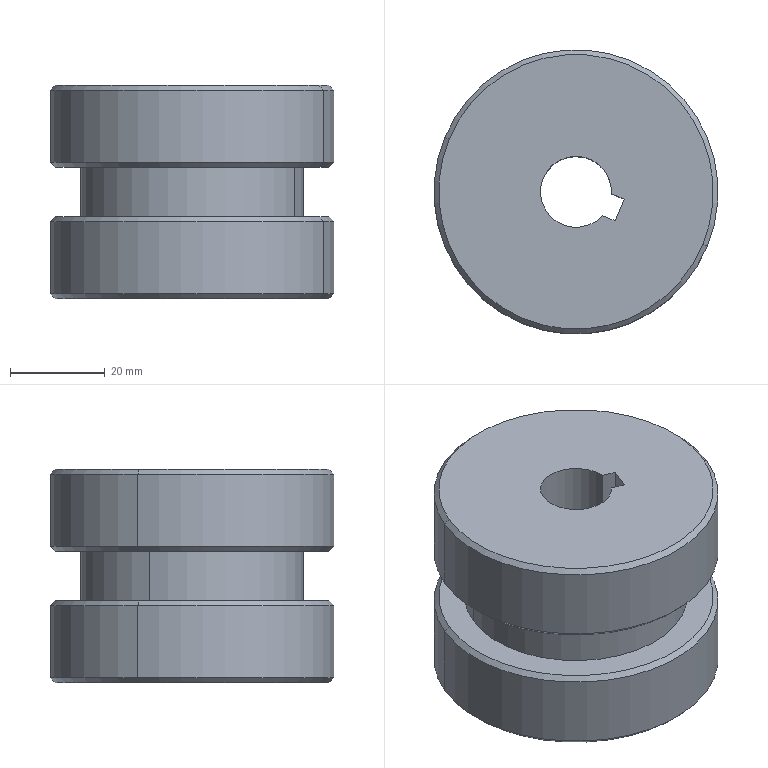Component | SolidWorks | 170423A4-ConveyorSynchronousPulleyAssembly-1_170423A4-Pulley2-1 | 1 solid | 23 faces | box 60 x 60 x 45 mm | volume 106844 mm3 | cylinder 8 | cone 8 | plane 7 | commonest cylinder face diameters 60 x4 15 x2 47 x2
build123d program:
from build123d import *

# Parameters (mm, degrees)
SKETCH1_R           = 30
BOSS_EXTRUDE1_DEPTH = 22.5
SKETCH5_W           = 6.5
SKETCH5_H           = 10.5
CHAMFER1_SIZE       = 1
SKETCH2_R           = 7.5
CUT_EXTRUDE1_DEPTH  = 62.847
SKETCH7_W           = 10
SKETCH7_H           = 5
CUT_EXTRUDE2_DEPTH  = 62.847


with BuildPart() as part:
    # Sketch1 → Boss-Extrude1 (new, symmetric)
    with BuildSketch(Plane.XY):
        with Locations(Location((0, 0, 0), (0, 0, 180))):
            Circle(SKETCH1_R)
    extrude(amount=BOSS_EXTRUDE1_DEPTH, both=True)

    # Sketch5 → Cut-Revolve1 (revolve, cut)
    with BuildSketch(Plane(origin=(0, 0, 0), x_dir=(1, 0, 0), z_dir=(0, 1, 0))):
        with Locations((-26.75, 0)):
            Rectangle(SKETCH5_W, SKETCH5_H)
    revolve(axis=Axis((0, 0, 0), (0, 0, 1)), mode=Mode.SUBTRACT)

    # Chamfer1
    chamfer1_edges = [part.edges().sort_by_distance(p)[0] for p in [
        (30, 0, -22.5),
        (30, 0, 22.5),
        (30, 0, 5.25),
        (30, 0, -5.25),
    ]]
    chamfer(chamfer1_edges, length=CHAMFER1_SIZE)

    # Sketch2 → Cut-Extrude1 (cut, through all)
    with BuildSketch(Plane.XY.offset(22.5)):
        Circle(SKETCH2_R)
    extrude(amount=-CUT_EXTRUDE1_DEPTH, mode=Mode.SUBTRACT)

    # Sketch7 → Cut-Extrude2 (cut, through all)
    with BuildSketch(Plane.XY.offset(22.5)):
        with Locations((-5, 0)):
            Rectangle(SKETCH7_W, SKETCH7_H)
    extrude(amount=-CUT_EXTRUDE2_DEPTH, mode=Mode.SUBTRACT)


solid = part.part

# Placed as in the assembly
solid = solid.moved(Location((99.754, -120.788, 444), (0, 0, 157.477)))
STEP:
#1=COLOUR_RGB('',0.7922,0.8196,0.9333);
#2=FILL_AREA_STYLE_COLOUR('',#1);
#3=FILL_AREA_STYLE('',(#2));
#4=SURFACE_STYLE_FILL_AREA(#3);
#5=SURFACE_SIDE_STYLE('',(#4));
#6=SURFACE_STYLE_USAGE(.BOTH.,#5);
#7=PRESENTATION_STYLE_ASSIGNMENT((#6));
#8=CARTESIAN_POINT('',(3.655,-4.642,16.594));
#9=VERTEX_POINT('',#8);
#10=CARTESIAN_POINT('',(4.147,-4.953,16.594));
#11=VERTEX_POINT('',#10);
#12=CARTESIAN_POINT('',(3.927,-4.755,16.594));
#13=DIRECTION('',(0.,-0.,1.));
#14=DIRECTION('',(-0.9237,0.383,0.));
#15=AXIS2_PLACEMENT_3D('',#12,#13,#14);
#16=CIRCLE('',#15,0.2953);
#17=EDGE_CURVE('',#9,#11,#16,.T.);
#18=ORIENTED_EDGE('',*,*,#17,.F.);
#19=CARTESIAN_POINT('',(3.655,-4.642,18.366));
#20=VERTEX_POINT('',#19);
#21=CARTESIAN_POINT('',(3.655,-4.642,16.594));
#22=DIRECTION('',(0.,-0.,1.));
#23=VECTOR('',#22,39.37);
#24=LINE('',#21,#23);
#25=EDGE_CURVE('',#9,#20,#24,.T.);
#26=ORIENTED_EDGE('',*,*,#25,.T.);
#27=CARTESIAN_POINT('',(4.147,-4.953,18.366));
#28=VERTEX_POINT('',#27);
#29=CARTESIAN_POINT('',(3.927,-4.755,18.366));
#30=DIRECTION('',(0.,-0.,1.));
#31=DIRECTION('',(-0.9237,0.383,0.));
#32=AXIS2_PLACEMENT_3D('',#29,#30,#31);
#33=CIRCLE('',#32,0.2953);
#34=EDGE_CURVE('',#20,#28,#33,.T.);
#35=ORIENTED_EDGE('',*,*,#34,.T.);
#36=CARTESIAN_POINT('',(4.147,-4.953,16.594));
#37=DIRECTION('',(-0.,0.,-1.));
#38=VECTOR('',#37,39.37);
#39=LINE('',#36,#38);
#40=EDGE_CURVE('',#28,#11,#39,.T.);
#41=ORIENTED_EDGE('',*,*,#40,.T.);
#42=EDGE_LOOP('',(#18,#26,#35,#41));
#43=FACE_OUTER_BOUND('',#42,.T.);
#44=CARTESIAN_POINT('',(3.927,-4.755,16.594));
#45=DIRECTION('',(0.,-0.,1.));
#46=DIRECTION('',(-0.9237,0.383,0.));
#47=AXIS2_PLACEMENT_3D('',#44,#45,#46);
#48=CYLINDRICAL_SURFACE('',#47,0.2953);
#49=ADVANCED_FACE('',(#43),#48,.F.);
#50=CARTESIAN_POINT('',(2.873,-4.318,18.366));
#51=VERTEX_POINT('',#50);
#52=CARTESIAN_POINT('',(4.982,-5.193,18.366));
#53=VERTEX_POINT('',#52);
#54=CARTESIAN_POINT('',(3.927,-4.755,18.366));
#55=DIRECTION('',(0.,-0.,1.));
#56=DIRECTION('',(-0.9237,0.383,0.));
#57=AXIS2_PLACEMENT_3D('',#54,#55,#56);
#58=CIRCLE('',#57,1.142);
#59=EDGE_CURVE('',#51,#53,#58,.T.);
#60=ORIENTED_EDGE('',*,*,#59,.F.);
#61=CARTESIAN_POINT('',(2.836,-4.303,18.327));
#62=VERTEX_POINT('',#61);
#63=CARTESIAN_POINT('',(2.873,-4.318,18.366));
#64=DIRECTION('',(-0.6532,0.2709,-0.7071));
#65=VECTOR('',#64,39.37);
#66=LINE('',#63,#65);
#67=EDGE_CURVE('',#51,#62,#66,.T.);
#68=ORIENTED_EDGE('',*,*,#67,.T.);
#69=CARTESIAN_POINT('',(5.018,-5.208,18.327));
#70=VERTEX_POINT('',#69);
#71=CARTESIAN_POINT('',(3.927,-4.755,18.327));
#72=DIRECTION('',(-0.,0.,-1.));
#73=DIRECTION('',(-0.9237,0.383,0.));
#74=AXIS2_PLACEMENT_3D('',#71,#72,#73);
#75=CIRCLE('',#74,1.181);
#76=EDGE_CURVE('',#70,#62,#75,.T.);
#77=ORIENTED_EDGE('',*,*,#76,.F.);
#78=CARTESIAN_POINT('',(4.982,-5.193,18.366));
#79=DIRECTION('',(0.6532,-0.2709,-0.7071));
#80=VECTOR('',#79,39.37);
#81=LINE('',#78,#80);
#82=EDGE_CURVE('',#53,#70,#81,.T.);
#83=ORIENTED_EDGE('',*,*,#82,.F.);
#84=EDGE_LOOP('',(#60,#68,#77,#83));
#85=FACE_OUTER_BOUND('',#84,.T.);
#86=CARTESIAN_POINT('',(3.927,-4.755,18.366));
#87=DIRECTION('',(-0.,0.,-1.));
#88=DIRECTION('',(0.9237,-0.383,-0.));
#89=AXIS2_PLACEMENT_3D('',#86,#87,#88);
#90=CONICAL_SURFACE('',#89,1.142,0.7854);
#91=ADVANCED_FACE('',(#85),#90,.T.);
#92=CARTESIAN_POINT('',(4.982,-5.193,17.687));
#93=VERTEX_POINT('',#92);
#94=CARTESIAN_POINT('',(2.873,-4.318,17.687));
#95=VERTEX_POINT('',#94);
#96=CARTESIAN_POINT('',(3.927,-4.755,17.687));
#97=DIRECTION('',(0.,0.,-1.));
#98=DIRECTION('',(-0.9237,0.383,0.));
#99=AXIS2_PLACEMENT_3D('',#96,#97,#98);
#100=CIRCLE('',#99,1.142);
#101=EDGE_CURVE('',#93,#95,#100,.T.);
#102=ORIENTED_EDGE('',*,*,#101,.F.);
#103=CARTESIAN_POINT('',(5.018,-5.208,17.726));
#104=VERTEX_POINT('',#103);
#105=CARTESIAN_POINT('',(4.982,-5.193,17.687));
#106=DIRECTION('',(0.6532,-0.2709,0.7071));
#107=VECTOR('',#106,39.37);
#108=LINE('',#105,#107);
#109=EDGE_CURVE('',#93,#104,#108,.T.);
#110=ORIENTED_EDGE('',*,*,#109,.T.);
#111=CARTESIAN_POINT('',(2.836,-4.303,17.726));
#112=VERTEX_POINT('',#111);
#113=CARTESIAN_POINT('',(3.927,-4.755,17.726));
#114=DIRECTION('',(0.,-0.,1.));
#115=DIRECTION('',(-0.9237,0.383,0.));
#116=AXIS2_PLACEMENT_3D('',#113,#114,#115);
#117=CIRCLE('',#116,1.181);
#118=EDGE_CURVE('',#112,#104,#117,.T.);
#119=ORIENTED_EDGE('',*,*,#118,.F.);
#120=CARTESIAN_POINT('',(2.873,-4.318,17.687));
#121=DIRECTION('',(-0.6532,0.2709,0.7071));
#122=VECTOR('',#121,39.37);
#123=LINE('',#120,#122);
#124=EDGE_CURVE('',#95,#112,#123,.T.);
#125=ORIENTED_EDGE('',*,*,#124,.F.);
#126=EDGE_LOOP('',(#102,#110,#119,#125));
#127=FACE_OUTER_BOUND('',#126,.T.);
#128=CARTESIAN_POINT('',(3.927,-4.755,17.687));
#129=DIRECTION('',(0.,-0.,1.));
#130=DIRECTION('',(-0.9237,0.383,0.));
#131=AXIS2_PLACEMENT_3D('',#128,#129,#130);
#132=CONICAL_SURFACE('',#131,1.142,0.7854);
#133=ADVANCED_FACE('',(#127),#132,.T.);
#134=CARTESIAN_POINT('',(2.873,-4.318,17.274));
#135=VERTEX_POINT('',#134);
#136=CARTESIAN_POINT('',(4.982,-5.193,17.274));
#137=VERTEX_POINT('',#136);
#138=CARTESIAN_POINT('',(3.927,-4.755,17.274));
#139=DIRECTION('',(-0.,-0.,1.));
#140=DIRECTION('',(0.9237,-0.383,-0.));
#141=AXIS2_PLACEMENT_3D('',#138,#139,#140);
#142=CIRCLE('',#141,1.142);
#143=EDGE_CURVE('',#135,#137,#142,.T.);
#144=ORIENTED_EDGE('',*,*,#143,.F.);
#145=CARTESIAN_POINT('',(2.836,-4.303,17.234));
#146=VERTEX_POINT('',#145);
#147=CARTESIAN_POINT('',(2.836,-4.303,17.234));
#148=DIRECTION('',(-0.6532,0.2709,-0.7071));
#149=VECTOR('',#148,39.37);
#150=LINE('',#147,#149);
#151=EDGE_CURVE('',#135,#146,#150,.T.);
#152=ORIENTED_EDGE('',*,*,#151,.T.);
#153=CARTESIAN_POINT('',(5.018,-5.208,17.234));
#154=VERTEX_POINT('',#153);
#155=CARTESIAN_POINT('',(3.927,-4.755,17.234));
#156=DIRECTION('',(-0.,0.,-1.));
#157=DIRECTION('',(0.9237,-0.383,-0.));
#158=AXIS2_PLACEMENT_3D('',#155,#156,#157);
#159=CIRCLE('',#158,1.181);
#160=EDGE_CURVE('',#154,#146,#159,.T.);
#161=ORIENTED_EDGE('',*,*,#160,.F.);
#162=CARTESIAN_POINT('',(5.018,-5.208,17.234));
#163=DIRECTION('',(0.6532,-0.2709,-0.7071));
#164=VECTOR('',#163,39.37);
#165=LINE('',#162,#164);
#166=EDGE_CURVE('',#137,#154,#165,.T.);
#167=ORIENTED_EDGE('',*,*,#166,.F.);
#168=EDGE_LOOP('',(#144,#152,#161,#167));
#169=FACE_OUTER_BOUND('',#168,.T.);
#170=CARTESIAN_POINT('',(3.927,-4.755,17.234));
#171=DIRECTION('',(-0.,0.,-1.));
#172=DIRECTION('',(0.9237,-0.383,-0.));
#173=AXIS2_PLACEMENT_3D('',#170,#171,#172);
#174=CONICAL_SURFACE('',#173,1.181,0.7854);
#175=ADVANCED_FACE('',(#169),#174,.T.);
#176=CARTESIAN_POINT('',(4.982,-5.193,16.594));
#177=VERTEX_POINT('',#176);
#178=CARTESIAN_POINT('',(2.873,-4.318,16.594));
#179=VERTEX_POINT('',#178);
#180=CARTESIAN_POINT('',(3.927,-4.755,16.594));
#181=DIRECTION('',(-0.,0.,-1.));
#182=DIRECTION('',(-0.9237,0.383,0.));
#183=AXIS2_PLACEMENT_3D('',#180,#181,#182);
#184=CIRCLE('',#183,1.142);
#185=EDGE_CURVE('',#177,#179,#184,.T.);
#186=ORIENTED_EDGE('',*,*,#185,.F.);
#187=CARTESIAN_POINT('',(5.018,-5.208,16.634));
#188=VERTEX_POINT('',#187);
#189=CARTESIAN_POINT('',(5.018,-5.208,16.634));
#190=DIRECTION('',(0.6532,-0.2709,0.7071));
#191=VECTOR('',#190,39.37);
#192=LINE('',#189,#191);
#193=EDGE_CURVE('',#177,#188,#192,.T.);
#194=ORIENTED_EDGE('',*,*,#193,.T.);
#195=CARTESIAN_POINT('',(2.836,-4.303,16.634));
#196=VERTEX_POINT('',#195);
#197=CARTESIAN_POINT('',(3.927,-4.755,16.634));
#198=DIRECTION('',(0.,-0.,1.));
#199=DIRECTION('',(-0.9237,0.383,0.));
#200=AXIS2_PLACEMENT_3D('',#197,#198,#199);
#201=CIRCLE('',#200,1.181);
#202=EDGE_CURVE('',#196,#188,#201,.T.);
#203=ORIENTED_EDGE('',*,*,#202,.F.);
#204=CARTESIAN_POINT('',(2.836,-4.303,16.634));
#205=DIRECTION('',(-0.6532,0.2709,0.7071));
#206=VECTOR('',#205,39.37);
#207=LINE('',#204,#206);
#208=EDGE_CURVE('',#179,#196,#207,.T.);
#209=ORIENTED_EDGE('',*,*,#208,.F.);
#210=EDGE_LOOP('',(#186,#194,#203,#209));
#211=FACE_OUTER_BOUND('',#210,.T.);
#212=CARTESIAN_POINT('',(3.927,-4.755,16.634));
#213=DIRECTION('',(0.,-0.,1.));
#214=DIRECTION('',(-0.9237,0.383,0.));
#215=AXIS2_PLACEMENT_3D('',#212,#213,#214);
#216=CONICAL_SURFACE('',#215,1.181,0.7854);
#217=ADVANCED_FACE('',(#211),#216,.T.);
#218=ORIENTED_EDGE('',*,*,#160,.T.);
#219=CARTESIAN_POINT('',(2.836,-4.303,18.366));
#220=DIRECTION('',(-0.,0.,-1.));
#221=VECTOR('',#220,39.37);
#222=LINE('',#219,#221);
#223=EDGE_CURVE('',#146,#196,#222,.T.);
#224=ORIENTED_EDGE('',*,*,#223,.T.);
#225=ORIENTED_EDGE('',*,*,#202,.T.);
#226=CARTESIAN_POINT('',(5.018,-5.208,18.366));
#227=DIRECTION('',(-0.,0.,-1.));
#228=VECTOR('',#227,39.37);
#229=LINE('',#226,#228);
#230=EDGE_CURVE('',#154,#188,#229,.T.);
#231=ORIENTED_EDGE('',*,*,#230,.F.);
#232=EDGE_LOOP('',(#218,#224,#225,#231));
#233=FACE_OUTER_BOUND('',#232,.T.);
#234=CARTESIAN_POINT('',(3.927,-4.755,18.366));
#235=DIRECTION('',(-0.,0.,-1.));
#236=DIRECTION('',(0.9237,-0.383,-0.));
#237=AXIS2_PLACEMENT_3D('',#234,#235,#236);
#238=CYLINDRICAL_SURFACE('',#237,1.181);
#239=ADVANCED_FACE('',(#233),#238,.T.);
#240=CARTESIAN_POINT('',(4.782,-5.11,17.687));
#241=VERTEX_POINT('',#240);
#242=CARTESIAN_POINT('',(3.073,-4.401,17.687));
#243=VERTEX_POINT('',#242);
#244=CARTESIAN_POINT('',(3.927,-4.755,17.687));
#245=DIRECTION('',(0.,0.,-1.));
#246=DIRECTION('',(0.9237,-0.383,-0.));
#247=AXIS2_PLACEMENT_3D('',#244,#245,#246);
#248=CIRCLE('',#247,0.9252);
#249=EDGE_CURVE('',#241,#243,#248,.T.);
#250=ORIENTED_EDGE('',*,*,#249,.T.);
#251=CARTESIAN_POINT('',(3.073,-4.401,17.274));
#252=VERTEX_POINT('',#251);
#253=CARTESIAN_POINT('',(3.073,-4.401,17.48));
#254=DIRECTION('',(0.,0.,-1.));
#255=VECTOR('',#254,39.37);
#256=LINE('',#253,#255);
#257=EDGE_CURVE('',#243,#252,#256,.T.);
#258=ORIENTED_EDGE('',*,*,#257,.T.);
#259=CARTESIAN_POINT('',(4.782,-5.11,17.274));
#260=VERTEX_POINT('',#259);
#261=CARTESIAN_POINT('',(3.927,-4.755,17.274));
#262=DIRECTION('',(0.,0.,-1.));
#263=DIRECTION('',(0.9237,-0.383,-0.));
#264=AXIS2_PLACEMENT_3D('',#261,#262,#263);
#265=CIRCLE('',#264,0.9252);
#266=EDGE_CURVE('',#260,#252,#265,.T.);
#267=ORIENTED_EDGE('',*,*,#266,.F.);
#268=CARTESIAN_POINT('',(4.782,-5.11,17.48));
#269=DIRECTION('',(0.,0.,-1.));
#270=VECTOR('',#269,39.37);
#271=LINE('',#268,#270);
#272=EDGE_CURVE('',#241,#260,#271,.T.);
#273=ORIENTED_EDGE('',*,*,#272,.F.);
#274=EDGE_LOOP('',(#250,#258,#267,#273));
#275=FACE_OUTER_BOUND('',#274,.T.);
#276=CARTESIAN_POINT('',(3.927,-4.755,17.48));
#277=DIRECTION('',(0.,0.,-1.));
#278=DIRECTION('',(0.9237,-0.383,-0.));
#279=AXIS2_PLACEMENT_3D('',#276,#277,#278);
#280=CYLINDRICAL_SURFACE('',#279,0.9252);
#281=ADVANCED_FACE('',(#275),#280,.T.);
#282=ORIENTED_EDGE('',*,*,#76,.T.);
#283=CARTESIAN_POINT('',(2.836,-4.303,18.366));
#284=DIRECTION('',(-0.,0.,-1.));
#285=VECTOR('',#284,39.37);
#286=LINE('',#283,#285);
#287=EDGE_CURVE('',#62,#112,#286,.T.);
#288=ORIENTED_EDGE('',*,*,#287,.T.);
#289=ORIENTED_EDGE('',*,*,#118,.T.);
#290=CARTESIAN_POINT('',(5.018,-5.208,18.366));
#291=DIRECTION('',(-0.,0.,-1.));
#292=VECTOR('',#291,39.37);
#293=LINE('',#290,#292);
#294=EDGE_CURVE('',#70,#104,#293,.T.);
#295=ORIENTED_EDGE('',*,*,#294,.F.);
#296=EDGE_LOOP('',(#282,#288,#289,#295));
#297=FACE_OUTER_BOUND('',#296,.T.);
#298=CARTESIAN_POINT('',(3.927,-4.755,18.366));
#299=DIRECTION('',(-0.,0.,-1.));
#300=DIRECTION('',(0.9237,-0.383,-0.));
#301=AXIS2_PLACEMENT_3D('',#298,#299,#300);
#302=CYLINDRICAL_SURFACE('',#301,1.181);
#303=ADVANCED_FACE('',(#297),#302,.T.);
#304=ORIENTED_EDGE('',*,*,#287,.F.);
#305=CARTESIAN_POINT('',(3.927,-4.755,18.327));
#306=DIRECTION('',(-0.,0.,-1.));
#307=DIRECTION('',(-0.9237,0.383,0.));
#308=AXIS2_PLACEMENT_3D('',#305,#306,#307);
#309=CIRCLE('',#308,1.181);
#310=EDGE_CURVE('',#62,#70,#309,.T.);
#311=ORIENTED_EDGE('',*,*,#310,.T.);
#312=ORIENTED_EDGE('',*,*,#294,.T.);
#313=CARTESIAN_POINT('',(3.927,-4.755,17.726));
#314=DIRECTION('',(0.,-0.,1.));
#315=DIRECTION('',(-0.9237,0.383,0.));
#316=AXIS2_PLACEMENT_3D('',#313,#314,#315);
#317=CIRCLE('',#316,1.181);
#318=EDGE_CURVE('',#104,#112,#317,.T.);
#319=ORIENTED_EDGE('',*,*,#318,.T.);
#320=EDGE_LOOP('',(#304,#311,#312,#319));
#321=FACE_OUTER_BOUND('',#320,.T.);
#322=CARTESIAN_POINT('',(3.927,-4.755,18.366));
#323=DIRECTION('',(-0.,0.,-1.));
#324=DIRECTION('',(0.9237,-0.383,-0.));
#325=AXIS2_PLACEMENT_3D('',#322,#323,#324);
#326=CYLINDRICAL_SURFACE('',#325,1.181);
#327=ADVANCED_FACE('',(#321),#326,.T.);
#328=CARTESIAN_POINT('',(4.329,-4.815,18.366));
#329=VERTEX_POINT('',#328);
#330=CARTESIAN_POINT('',(4.222,-4.771,18.366));
#331=VERTEX_POINT('',#330);
#332=CARTESIAN_POINT('',(3.965,-4.665,18.366));
#333=DIRECTION('',(-0.9237,0.383,0.));
#334=VECTOR('',#333,39.37);
#335=LINE('',#332,#334);
#336=EDGE_CURVE('',#329,#331,#335,.T.);
#337=ORIENTED_EDGE('',*,*,#336,.F.);
#338=CARTESIAN_POINT('',(4.253,-4.997,18.366));
#339=VERTEX_POINT('',#338);
#340=CARTESIAN_POINT('',(4.329,-4.815,18.366));
#341=DIRECTION('',(0.383,0.9237,0.));
#342=VECTOR('',#341,39.37);
#343=LINE('',#340,#342);
#344=EDGE_CURVE('',#339,#329,#343,.T.);
#345=ORIENTED_EDGE('',*,*,#344,.F.);
#346=CARTESIAN_POINT('',(3.89,-4.846,18.366));
#347=DIRECTION('',(0.9237,-0.383,-0.));
#348=VECTOR('',#347,39.37);
#349=LINE('',#346,#348);
#350=EDGE_CURVE('',#28,#339,#349,.T.);
#351=ORIENTED_EDGE('',*,*,#350,.F.);
#352=ORIENTED_EDGE('',*,*,#34,.F.);
#353=CARTESIAN_POINT('',(3.927,-4.755,18.366));
#354=DIRECTION('',(0.,-0.,1.));
#355=DIRECTION('',(-0.9237,0.383,0.));
#356=AXIS2_PLACEMENT_3D('',#353,#354,#355);
#357=CIRCLE('',#356,0.2953);
#358=EDGE_CURVE('',#331,#20,#357,.T.);
#359=ORIENTED_EDGE('',*,*,#358,.F.);
#360=EDGE_LOOP('',(#337,#345,#351,#352,#359));
#361=FACE_BOUND('',#360,.T.);
#362=CARTESIAN_POINT('',(3.927,-4.755,18.366));
#363=DIRECTION('',(0.,-0.,1.));
#364=DIRECTION('',(-0.9237,0.383,0.));
#365=AXIS2_PLACEMENT_3D('',#362,#363,#364);
#366=CIRCLE('',#365,1.142);
#367=EDGE_CURVE('',#53,#51,#366,.T.);
#368=ORIENTED_EDGE('',*,*,#367,.T.);
#369=ORIENTED_EDGE('',*,*,#59,.T.);
#370=EDGE_LOOP('',(#368,#369));
#371=FACE_OUTER_BOUND('',#370,.T.);
#372=CARTESIAN_POINT('',(3.927,-4.755,18.366));
#373=DIRECTION('',(0.,-0.,1.));
#374=DIRECTION('',(-0.9237,0.383,0.));
#375=AXIS2_PLACEMENT_3D('',#372,#373,#374);
#376=PLANE('',#375);
#377=ADVANCED_FACE('',(#361,#371),#376,.T.);
#378=CARTESIAN_POINT('',(3.927,-4.755,17.687));
#379=DIRECTION('',(0.,0.,-1.));
#380=DIRECTION('',(-0.9237,0.383,0.));
#381=AXIS2_PLACEMENT_3D('',#378,#379,#380);
#382=CIRCLE('',#381,1.142);
#383=EDGE_CURVE('',#95,#93,#382,.T.);
#384=ORIENTED_EDGE('',*,*,#383,.T.);
#385=ORIENTED_EDGE('',*,*,#101,.T.);
#386=EDGE_LOOP('',(#384,#385));
#387=FACE_OUTER_BOUND('',#386,.T.);
#388=ORIENTED_EDGE('',*,*,#249,.F.);
#389=CARTESIAN_POINT('',(3.927,-4.755,17.687));
#390=DIRECTION('',(0.,0.,-1.));
#391=DIRECTION('',(0.9237,-0.383,-0.));
#392=AXIS2_PLACEMENT_3D('',#389,#390,#391);
#393=CIRCLE('',#392,0.9252);
#394=EDGE_CURVE('',#243,#241,#393,.T.);
#395=ORIENTED_EDGE('',*,*,#394,.F.);
#396=EDGE_LOOP('',(#388,#395));
#397=FACE_BOUND('',#396,.T.);
#398=CARTESIAN_POINT('',(5.018,-5.208,17.687));
#399=DIRECTION('',(-0.,-0.,1.));
#400=DIRECTION('',(-0.9237,0.383,0.));
#401=AXIS2_PLACEMENT_3D('',#398,#399,#400);
#402=PLANE('',#401);
#403=ADVANCED_FACE('',(#387,#397),#402,.F.);
#404=ORIENTED_EDGE('',*,*,#257,.F.);
#405=ORIENTED_EDGE('',*,*,#394,.T.);
#406=ORIENTED_EDGE('',*,*,#272,.T.);
#407=CARTESIAN_POINT('',(3.927,-4.755,17.274));
#408=DIRECTION('',(0.,0.,-1.));
#409=DIRECTION('',(0.9237,-0.383,-0.));
#410=AXIS2_PLACEMENT_3D('',#407,#408,#409);
#411=CIRCLE('',#410,0.9252);
#412=EDGE_CURVE('',#252,#260,#411,.T.);
#413=ORIENTED_EDGE('',*,*,#412,.F.);
#414=EDGE_LOOP('',(#404,#405,#406,#413));
#415=FACE_OUTER_BOUND('',#414,.T.);
#416=CARTESIAN_POINT('',(3.927,-4.755,17.48));
#417=DIRECTION('',(0.,0.,-1.));
#418=DIRECTION('',(0.9237,-0.383,-0.));
#419=AXIS2_PLACEMENT_3D('',#416,#417,#418);
#420=CYLINDRICAL_SURFACE('',#419,0.9252);
#421=ADVANCED_FACE('',(#415),#420,.T.);
#422=CARTESIAN_POINT('',(3.927,-4.755,17.274));
#423=DIRECTION('',(-0.,-0.,1.));
#424=DIRECTION('',(0.9237,-0.383,-0.));
#425=AXIS2_PLACEMENT_3D('',#422,#423,#424);
#426=CIRCLE('',#425,1.142);
#427=EDGE_CURVE('',#137,#135,#426,.T.);
#428=ORIENTED_EDGE('',*,*,#427,.T.);
#429=ORIENTED_EDGE('',*,*,#143,.T.);
#430=EDGE_LOOP('',(#428,#429));
#431=FACE_OUTER_BOUND('',#430,.T.);
#432=ORIENTED_EDGE('',*,*,#266,.T.);
#433=ORIENTED_EDGE('',*,*,#412,.T.);
#434=EDGE_LOOP('',(#432,#433));
#435=FACE_BOUND('',#434,.T.);
#436=CARTESIAN_POINT('',(5.018,-5.208,17.274));
#437=DIRECTION('',(0.,0.,-1.));
#438=DIRECTION('',(0.9237,-0.383,-0.));
#439=AXIS2_PLACEMENT_3D('',#436,#437,#438);
#440=PLANE('',#439);
#441=ADVANCED_FACE('',(#431,#435),#440,.F.);
#442=CARTESIAN_POINT('',(4.253,-4.997,16.594));
#443=VERTEX_POINT('',#442);
#444=CARTESIAN_POINT('',(4.329,-4.815,16.594));
#445=VERTEX_POINT('',#444);
#446=CARTESIAN_POINT('',(4.329,-4.815,16.594));
#447=DIRECTION('',(0.383,0.9237,0.));
#448=VECTOR('',#447,39.37);
#449=LINE('',#446,#448);
#450=EDGE_CURVE('',#443,#445,#449,.T.);
#451=ORIENTED_EDGE('',*,*,#450,.T.);
#452=CARTESIAN_POINT('',(4.222,-4.771,16.594));
#453=VERTEX_POINT('',#452);
#454=CARTESIAN_POINT('',(3.965,-4.665,16.594));
#455=DIRECTION('',(-0.9237,0.383,0.));
#456=VECTOR('',#455,39.37);
#457=LINE('',#454,#456);
#458=EDGE_CURVE('',#445,#453,#457,.T.);
#459=ORIENTED_EDGE('',*,*,#458,.T.);
#460=CARTESIAN_POINT('',(3.927,-4.755,16.594));
#461=DIRECTION('',(0.,-0.,1.));
#462=DIRECTION('',(-0.9237,0.383,0.));
#463=AXIS2_PLACEMENT_3D('',#460,#461,#462);
#464=CIRCLE('',#463,0.2953);
#465=EDGE_CURVE('',#453,#9,#464,.T.);
#466=ORIENTED_EDGE('',*,*,#465,.T.);
#467=ORIENTED_EDGE('',*,*,#17,.T.);
#468=CARTESIAN_POINT('',(3.89,-4.846,16.594));
#469=DIRECTION('',(0.9237,-0.383,-0.));
#470=VECTOR('',#469,39.37);
#471=LINE('',#468,#470);
#472=EDGE_CURVE('',#11,#443,#471,.T.);
#473=ORIENTED_EDGE('',*,*,#472,.T.);
#474=EDGE_LOOP('',(#451,#459,#466,#467,#473));
#475=FACE_BOUND('',#474,.T.);
#476=CARTESIAN_POINT('',(3.927,-4.755,16.594));
#477=DIRECTION('',(-0.,0.,-1.));
#478=DIRECTION('',(-0.9237,0.383,0.));
#479=AXIS2_PLACEMENT_3D('',#476,#477,#478);
#480=CIRCLE('',#479,1.142);
#481=EDGE_CURVE('',#179,#177,#480,.T.);
#482=ORIENTED_EDGE('',*,*,#481,.T.);
#483=ORIENTED_EDGE('',*,*,#185,.T.);
#484=EDGE_LOOP('',(#482,#483));
#485=FACE_OUTER_BOUND('',#484,.T.);
#486=CARTESIAN_POINT('',(3.927,-4.755,16.594));
#487=DIRECTION('',(0.,-0.,1.));
#488=DIRECTION('',(-0.9237,0.383,0.));
#489=AXIS2_PLACEMENT_3D('',#486,#487,#488);
#490=PLANE('',#489);
#491=ADVANCED_FACE('',(#475,#485),#490,.F.);
#492=ORIENTED_EDGE('',*,*,#223,.F.);
#493=CARTESIAN_POINT('',(3.927,-4.755,17.234));
#494=DIRECTION('',(-0.,0.,-1.));
#495=DIRECTION('',(0.9237,-0.383,-0.));
#496=AXIS2_PLACEMENT_3D('',#493,#494,#495);
#497=CIRCLE('',#496,1.181);
#498=EDGE_CURVE('',#146,#154,#497,.T.);
#499=ORIENTED_EDGE('',*,*,#498,.T.);
#500=ORIENTED_EDGE('',*,*,#230,.T.);
#501=CARTESIAN_POINT('',(3.927,-4.755,16.634));
#502=DIRECTION('',(0.,-0.,1.));
#503=DIRECTION('',(-0.9237,0.383,0.));
#504=AXIS2_PLACEMENT_3D('',#501,#502,#503);
#505=CIRCLE('',#504,1.181);
#506=EDGE_CURVE('',#188,#196,#505,.T.);
#507=ORIENTED_EDGE('',*,*,#506,.T.);
#508=EDGE_LOOP('',(#492,#499,#500,#507));
#509=FACE_OUTER_BOUND('',#508,.T.);
#510=CARTESIAN_POINT('',(3.927,-4.755,18.366));
#511=DIRECTION('',(-0.,0.,-1.));
#512=DIRECTION('',(0.9237,-0.383,-0.));
#513=AXIS2_PLACEMENT_3D('',#510,#511,#512);
#514=CYLINDRICAL_SURFACE('',#513,1.181);
#515=ADVANCED_FACE('',(#509),#514,.T.);
#516=ORIENTED_EDGE('',*,*,#193,.F.);
#517=ORIENTED_EDGE('',*,*,#481,.F.);
#518=ORIENTED_EDGE('',*,*,#208,.T.);
#519=ORIENTED_EDGE('',*,*,#506,.F.);
#520=EDGE_LOOP('',(#516,#517,#518,#519));
#521=FACE_OUTER_BOUND('',#520,.T.);
#522=CARTESIAN_POINT('',(3.927,-4.755,16.634));
#523=DIRECTION('',(0.,-0.,1.));
#524=DIRECTION('',(-0.9237,0.383,0.));
#525=AXIS2_PLACEMENT_3D('',#522,#523,#524);
#526=CONICAL_SURFACE('',#525,1.181,0.7854);
#527=ADVANCED_FACE('',(#521),#526,.T.);
#528=ORIENTED_EDGE('',*,*,#151,.F.);
#529=ORIENTED_EDGE('',*,*,#427,.F.);
#530=ORIENTED_EDGE('',*,*,#166,.T.);
#531=ORIENTED_EDGE('',*,*,#498,.F.);
#532=EDGE_LOOP('',(#528,#529,#530,#531));
#533=FACE_OUTER_BOUND('',#532,.T.);
#534=CARTESIAN_POINT('',(3.927,-4.755,17.234));
#535=DIRECTION('',(-0.,0.,-1.));
#536=DIRECTION('',(0.9237,-0.383,-0.));
#537=AXIS2_PLACEMENT_3D('',#534,#535,#536);
#538=CONICAL_SURFACE('',#537,1.181,0.7854);
#539=ADVANCED_FACE('',(#533),#538,.T.);
#540=ORIENTED_EDGE('',*,*,#109,.F.);
#541=ORIENTED_EDGE('',*,*,#383,.F.);
#542=ORIENTED_EDGE('',*,*,#124,.T.);
#543=ORIENTED_EDGE('',*,*,#318,.F.);
#544=EDGE_LOOP('',(#540,#541,#542,#543));
#545=FACE_OUTER_BOUND('',#544,.T.);
#546=CARTESIAN_POINT('',(3.927,-4.755,17.687));
#547=DIRECTION('',(0.,-0.,1.));
#548=DIRECTION('',(-0.9237,0.383,0.));
#549=AXIS2_PLACEMENT_3D('',#546,#547,#548);
#550=CONICAL_SURFACE('',#549,1.142,0.7854);
#551=ADVANCED_FACE('',(#545),#550,.T.);
#552=ORIENTED_EDGE('',*,*,#67,.F.);
#553=ORIENTED_EDGE('',*,*,#367,.F.);
#554=ORIENTED_EDGE('',*,*,#82,.T.);
#555=ORIENTED_EDGE('',*,*,#310,.F.);
#556=EDGE_LOOP('',(#552,#553,#554,#555));
#557=FACE_OUTER_BOUND('',#556,.T.);
#558=CARTESIAN_POINT('',(3.927,-4.755,18.366));
#559=DIRECTION('',(-0.,0.,-1.));
#560=DIRECTION('',(0.9237,-0.383,-0.));
#561=AXIS2_PLACEMENT_3D('',#558,#559,#560);
#562=CONICAL_SURFACE('',#561,1.142,0.7854);
#563=ADVANCED_FACE('',(#557),#562,.T.);
#564=ORIENTED_EDGE('',*,*,#25,.F.);
#565=ORIENTED_EDGE('',*,*,#465,.F.);
#566=CARTESIAN_POINT('',(4.222,-4.771,16.594));
#567=DIRECTION('',(0.,-0.,1.));
#568=VECTOR('',#567,39.37);
#569=LINE('',#566,#568);
#570=EDGE_CURVE('',#453,#331,#569,.T.);
#571=ORIENTED_EDGE('',*,*,#570,.T.);
#572=ORIENTED_EDGE('',*,*,#358,.T.);
#573=EDGE_LOOP('',(#564,#565,#571,#572));
#574=FACE_OUTER_BOUND('',#573,.T.);
#575=CARTESIAN_POINT('',(3.927,-4.755,16.594));
#576=DIRECTION('',(0.,-0.,1.));
#577=DIRECTION('',(-0.9237,0.383,0.));
#578=AXIS2_PLACEMENT_3D('',#575,#576,#577);
#579=CYLINDRICAL_SURFACE('',#578,0.2953);
#580=ADVANCED_FACE('',(#574),#579,.F.);
#581=ORIENTED_EDGE('',*,*,#458,.F.);
#582=CARTESIAN_POINT('',(4.329,-4.815,16.594));
#583=DIRECTION('',(0.,-0.,1.));
#584=VECTOR('',#583,39.37);
#585=LINE('',#582,#584);
#586=EDGE_CURVE('',#445,#329,#585,.T.);
#587=ORIENTED_EDGE('',*,*,#586,.T.);
#588=ORIENTED_EDGE('',*,*,#336,.T.);
#589=ORIENTED_EDGE('',*,*,#570,.F.);
#590=EDGE_LOOP('',(#581,#587,#588,#589));
#591=FACE_OUTER_BOUND('',#590,.T.);
#592=CARTESIAN_POINT('',(3.965,-4.665,16.594));
#593=DIRECTION('',(0.383,0.9237,0.));
#594=DIRECTION('',(-0.9237,0.383,0.));
#595=AXIS2_PLACEMENT_3D('',#592,#593,#594);
#596=PLANE('',#595);
#597=ADVANCED_FACE('',(#591),#596,.F.);
#598=ORIENTED_EDGE('',*,*,#350,.T.);
#599=CARTESIAN_POINT('',(4.253,-4.997,16.594));
#600=DIRECTION('',(0.,-0.,1.));
#601=VECTOR('',#600,39.37);
#602=LINE('',#599,#601);
#603=EDGE_CURVE('',#443,#339,#602,.T.);
#604=ORIENTED_EDGE('',*,*,#603,.F.);
#605=ORIENTED_EDGE('',*,*,#472,.F.);
#606=ORIENTED_EDGE('',*,*,#40,.F.);
#607=EDGE_LOOP('',(#598,#604,#605,#606));
#608=FACE_OUTER_BOUND('',#607,.T.);
#609=CARTESIAN_POINT('',(3.89,-4.846,16.594));
#610=DIRECTION('',(-0.383,-0.9237,-0.));
#611=DIRECTION('',(0.9237,-0.383,-0.));
#612=AXIS2_PLACEMENT_3D('',#609,#610,#611);
#613=PLANE('',#612);
#614=ADVANCED_FACE('',(#608),#613,.F.);
#615=ORIENTED_EDGE('',*,*,#344,.T.);
#616=ORIENTED_EDGE('',*,*,#586,.F.);
#617=ORIENTED_EDGE('',*,*,#450,.F.);
#618=ORIENTED_EDGE('',*,*,#603,.T.);
#619=EDGE_LOOP('',(#615,#616,#617,#618));
#620=FACE_OUTER_BOUND('',#619,.T.);
#621=CARTESIAN_POINT('',(4.329,-4.815,16.594));
#622=DIRECTION('',(0.9237,-0.383,-0.));
#623=DIRECTION('',(0.,-0.,1.));
#624=AXIS2_PLACEMENT_3D('',#621,#622,#623);
#625=PLANE('',#624);
#626=ADVANCED_FACE('',(#620),#625,.F.);
#627=CLOSED_SHELL('',(#49,#91,#133,#175,#217,#239,#281,#303,#327,#377,#403,#421,#441,#491,#515,#527,#539,#551,#563,#580,#597,#614,#626));
#628=MANIFOLD_SOLID_BREP('',#627);
#629=STYLED_ITEM('',(#7),#628);
#630=(LENGTH_UNIT()NAMED_UNIT(*)SI_UNIT($,.METRE.));
#631=LENGTH_MEASURE_WITH_UNIT(LENGTH_MEASURE(0.0254),#630);
#632=DIMENSIONAL_EXPONENTS(1.,0.,0.,0.,0.,0.,0.);
#633=(CONVERSION_BASED_UNIT('',#631)LENGTH_UNIT()NAMED_UNIT(#632));
#634=UNCERTAINTY_MEASURE_WITH_UNIT(LENGTH_MEASURE(0.00001),#633,'','');
#635=(NAMED_UNIT(*)PLANE_ANGLE_UNIT()SI_UNIT($,.RADIAN.));
#636=(NAMED_UNIT(*)SI_UNIT($,.STERADIAN.)SOLID_ANGLE_UNIT());
#637=(GEOMETRIC_REPRESENTATION_CONTEXT(3)GLOBAL_UNCERTAINTY_ASSIGNED_CONTEXT((#634))GLOBAL_UNIT_ASSIGNED_CONTEXT((#633,#635,#636))REPRESENTATION_CONTEXT('',''));
#638=MECHANICAL_DESIGN_GEOMETRIC_PRESENTATION_REPRESENTATION('',(#629),#637);
#639=CARTESIAN_POINT('',(0.,0.,0.));
#640=DIRECTION('',(0.,0.,1.));
#641=DIRECTION('',(1.,0.,0.));
#642=AXIS2_PLACEMENT_3D('',#639,#640,#641);
#643=(LENGTH_UNIT()NAMED_UNIT(*)SI_UNIT($,.METRE.));
#644=LENGTH_MEASURE_WITH_UNIT(LENGTH_MEASURE(0.0254),#643);
#645=DIMENSIONAL_EXPONENTS(1.,0.,0.,0.,0.,0.,0.);
#646=(CONVERSION_BASED_UNIT('',#644)LENGTH_UNIT()NAMED_UNIT(#645));
#647=UNCERTAINTY_MEASURE_WITH_UNIT(LENGTH_MEASURE(0.00001),#646,'','');
#648=(NAMED_UNIT(*)PLANE_ANGLE_UNIT()SI_UNIT($,.RADIAN.));
#649=(NAMED_UNIT(*)SI_UNIT($,.STERADIAN.)SOLID_ANGLE_UNIT());
#650=(GEOMETRIC_REPRESENTATION_CONTEXT(3)GLOBAL_UNCERTAINTY_ASSIGNED_CONTEXT((#647))GLOBAL_UNIT_ASSIGNED_CONTEXT((#646,#648,#649))REPRESENTATION_CONTEXT('',''));
#651=ADVANCED_BREP_SHAPE_REPRESENTATION('',(#628,#642),#650);
#652=PRESENTATION_LAYER_ASSIGNMENT('','',(#629));